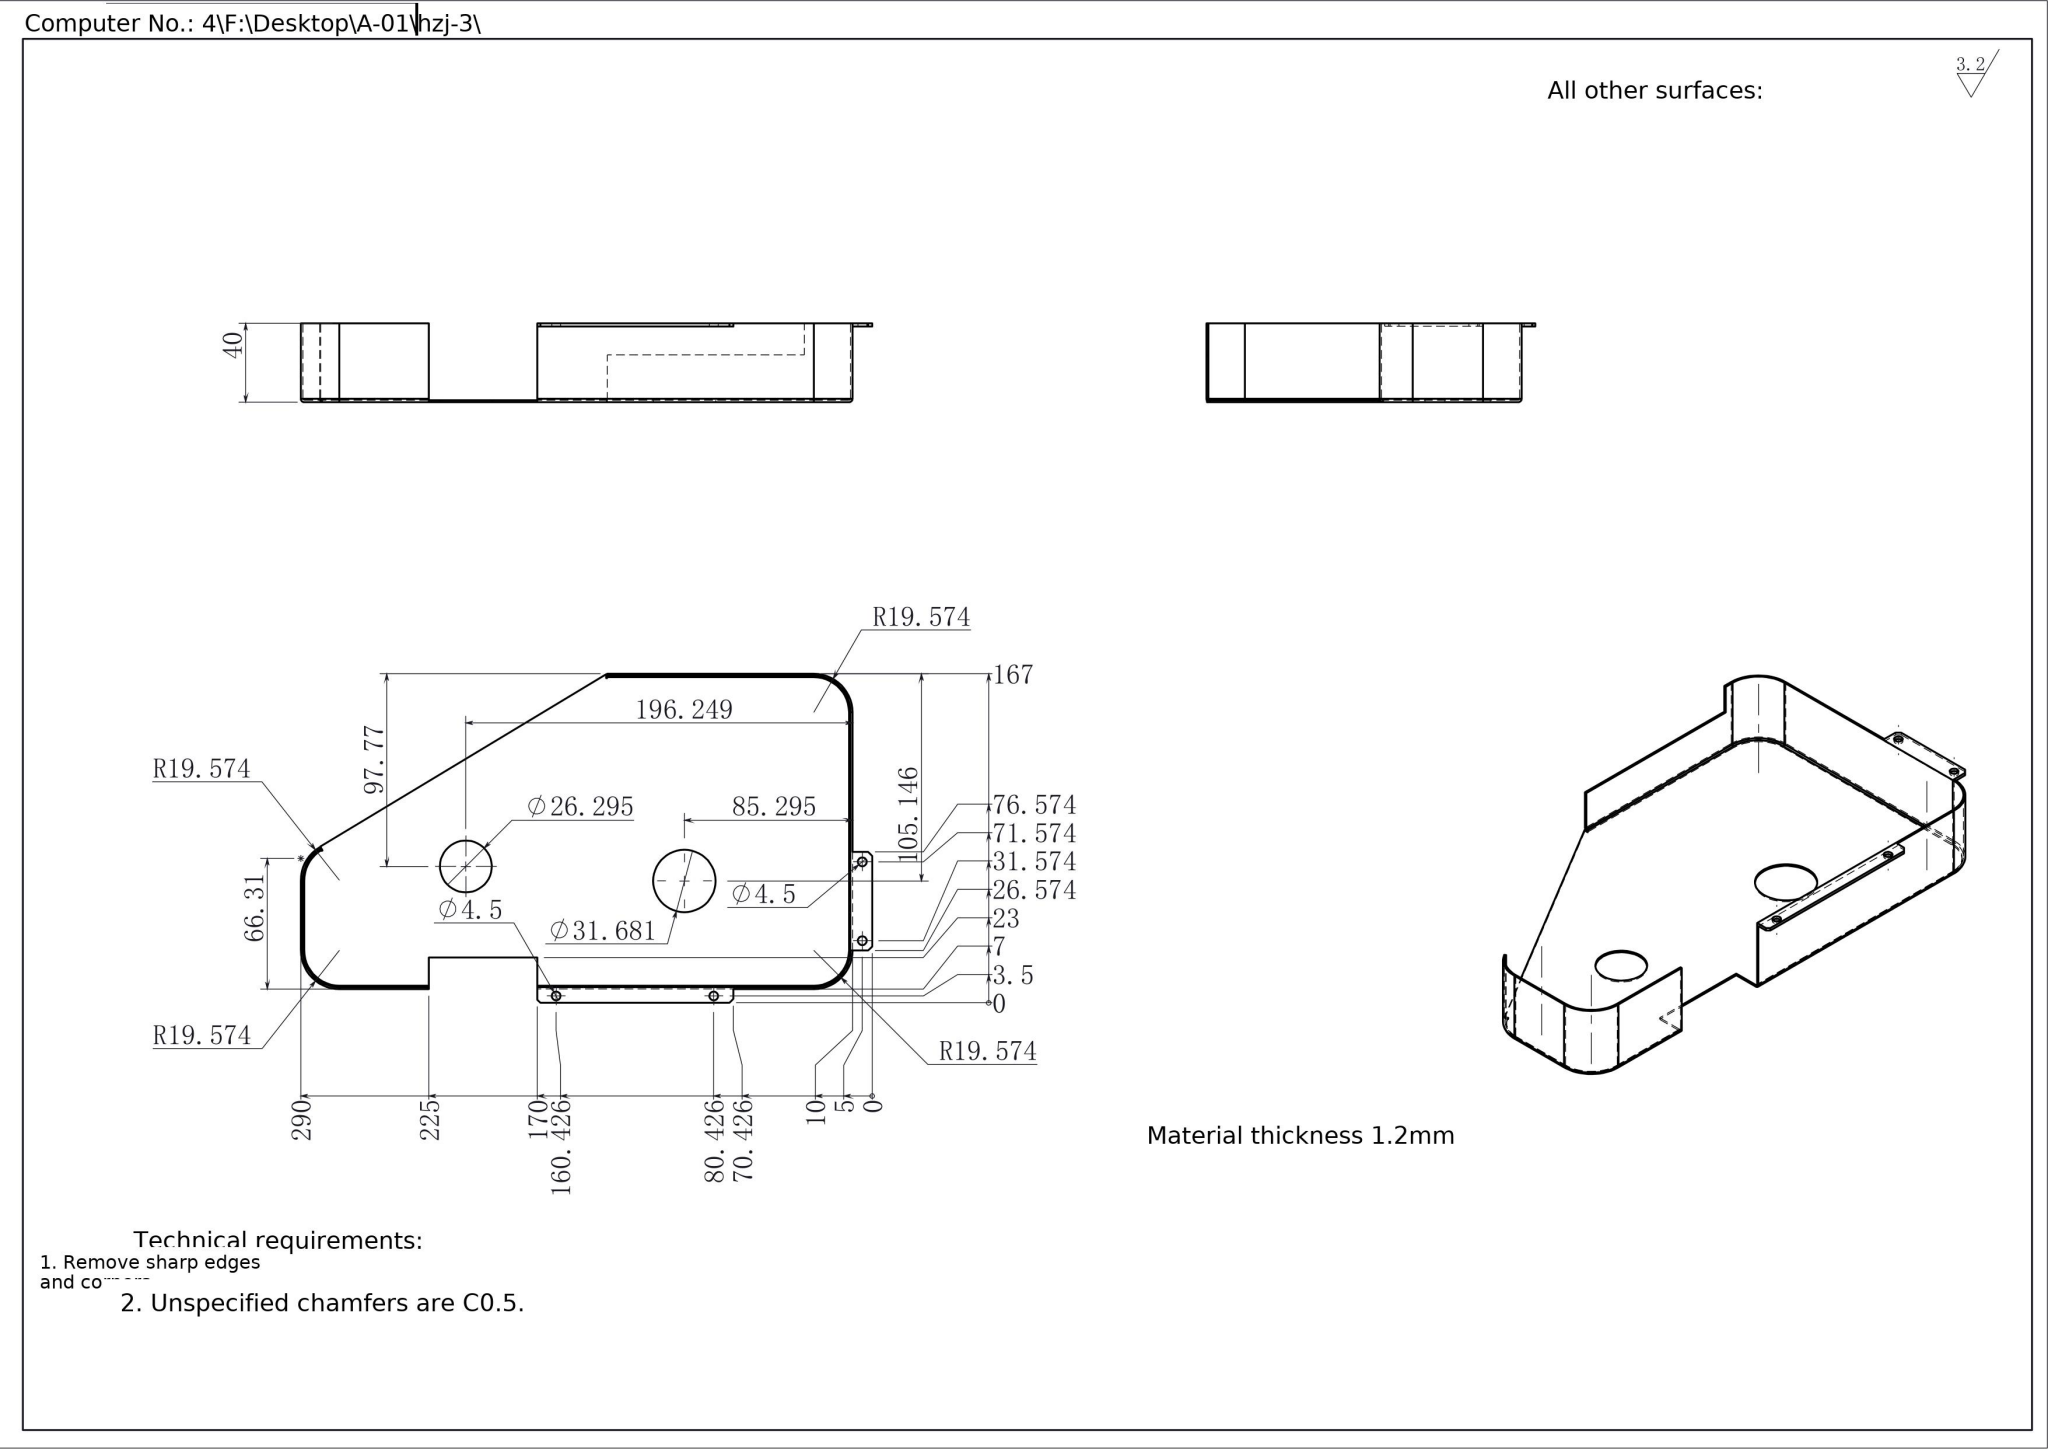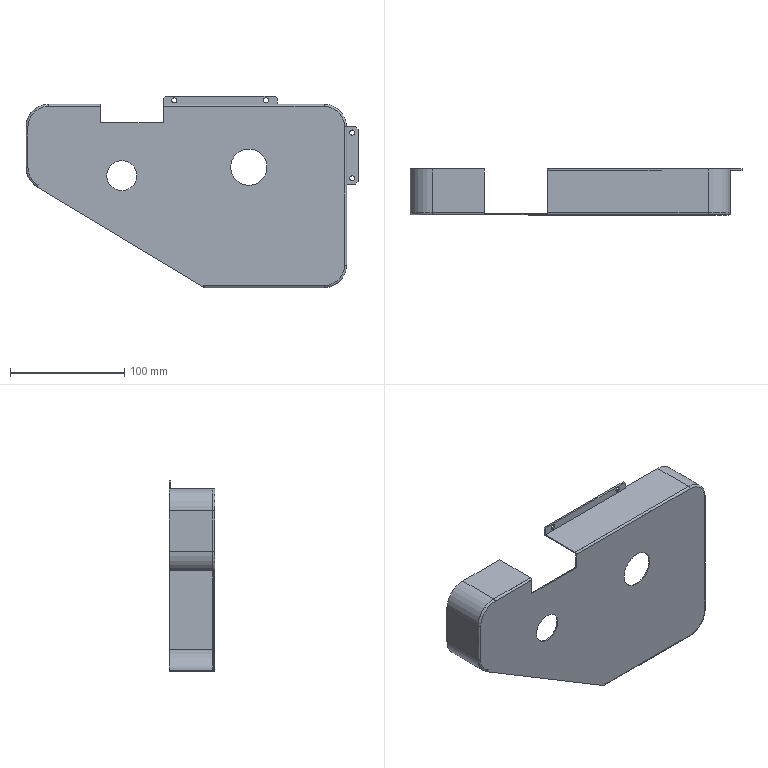Part | SolidWorks | mm | 1 solid | 86 faces | box 290 x 40 x 167 mm | volume 56543 mm3 | plane 48 | cylinder 30 | torus 8 | commonest cylinder face diameters 4.5 x8 1.473 x5 3.473 x5 37.147 x4 39.147 x4 31.681 x2 26.295 x2